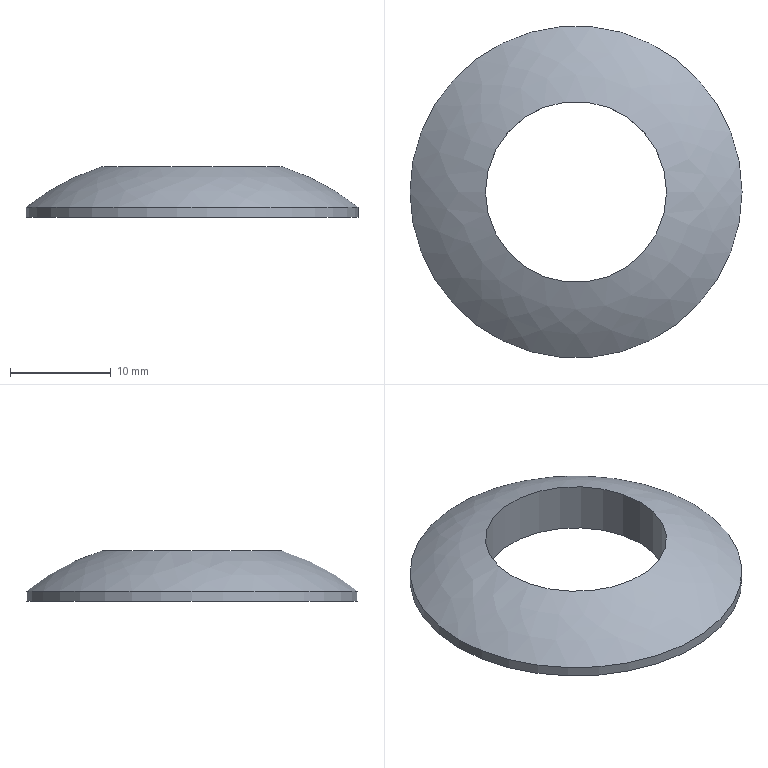Component | NX | SPHERICALWASHER2 | 1 solid | 4 faces | box 33 x 33 x 5 mm | volume 1856 mm3 | cylinder 2 | spline 1 | plane 1 | commonest cylinder face diameters 18 x1 33 x1
STEP:
#1=CARTESIAN_POINT('',(0.,0.,0.));
#2=DIRECTION('',(0.,0.,1.));
#3=DIRECTION('',(1.,0.,0.));
#4=AXIS2_PLACEMENT_3D('',#1,#2,#3);
#5=CARTESIAN_POINT('',(13.835,7.63,340.973));
#6=VERTEX_POINT('',#5);
#7=CARTESIAN_POINT('',(4.835,7.63,340.973));
#8=DIRECTION('',(0.,0.,-1.));
#9=DIRECTION('',(1.,0.,0.));
#10=AXIS2_PLACEMENT_3D('',#7,#8,#9);
#11=CIRCLE('',#10,9.);
#12=CARTESIAN_POINT('',(4.835,7.63,340.973));
#13=DIRECTION('',(0.,0.,-1.));
#14=DIRECTION('',(1.,0.,0.));
#15=AXIS2_PLACEMENT_3D('',#12,#13,#14);
#16=CYLINDRICAL_SURFACE('',#15,9.);
#17=CARTESIAN_POINT('',(0.,0.));
#18=DIRECTION('',(1.,0.));
#19=VECTOR('',#18,1.);
#20=LINE('',#17,#19);
#21=(GEOMETRIC_REPRESENTATION_CONTEXT(2)PARAMETRIC_REPRESENTATION_CONTEXT()REPRESENTATION_CONTEXT('',''));
#22=DEFINITIONAL_REPRESENTATION('',(#20),#21);
#23=PCURVE('',#16,#22);
#24=CARTESIAN_POINT('',(21.335,7.63,336.973));
#25=CARTESIAN_POINT('',(21.335,-25.37,336.973));
#26=CARTESIAN_POINT('',(-11.665,-25.37,336.973));
#27=CARTESIAN_POINT('',(-11.665,7.63,336.973));
#28=CARTESIAN_POINT('',(-11.665,40.63,336.973));
#29=CARTESIAN_POINT('',(21.335,40.63,336.973));
#30=CARTESIAN_POINT('',(21.335,7.63,336.973));
#31=CARTESIAN_POINT('',(19.087,7.63,338.746));
#32=CARTESIAN_POINT('',(19.087,-20.873,338.746));
#33=CARTESIAN_POINT('',(-9.417,-20.873,338.746));
#34=CARTESIAN_POINT('',(-9.417,7.63,338.746));
#35=CARTESIAN_POINT('',(-9.417,36.134,338.746));
#36=CARTESIAN_POINT('',(19.087,36.134,338.746));
#37=CARTESIAN_POINT('',(19.087,7.63,338.746));
#38=CARTESIAN_POINT('',(16.561,7.63,340.094));
#39=CARTESIAN_POINT('',(16.561,-15.82,340.094));
#40=CARTESIAN_POINT('',(-6.89,-15.82,340.094));
#41=CARTESIAN_POINT('',(-6.89,7.63,340.094));
#42=CARTESIAN_POINT('',(-6.89,31.081,340.094));
#43=CARTESIAN_POINT('',(16.561,31.081,340.094));
#44=CARTESIAN_POINT('',(16.561,7.63,340.094));
#45=CARTESIAN_POINT('',(13.835,7.63,340.973));
#46=CARTESIAN_POINT('',(13.835,-10.37,340.973));
#47=CARTESIAN_POINT('',(-4.165,-10.37,340.973));
#48=CARTESIAN_POINT('',(-4.165,7.63,340.973));
#49=CARTESIAN_POINT('',(-4.165,25.63,340.973));
#50=CARTESIAN_POINT('',(13.835,25.63,340.973));
#51=CARTESIAN_POINT('',(13.835,7.63,340.973));
#52=(BOUNDED_SURFACE()B_SPLINE_SURFACE(3,3,((#24,#25,#26,#27,#28,#29,#30),(#31,#32,#33,#34,#35,#36,#37),(#38,#39,#40,#41,#42,#43,#44),(#45,#46,#47,#48,#49,#50,#51)),.UNSPECIFIED.,.F.,.T.,.F.)B_SPLINE_SURFACE_WITH_KNOTS((4,4),(1,3,3,3,1),(0.,1.),(-0.5,0.,0.5,1.,1.5),.UNSPECIFIED.)GEOMETRIC_REPRESENTATION_ITEM()RATIONAL_B_SPLINE_SURFACE(((1.,0.3333,0.3333,1.,0.3333,0.3333,1.),(0.9895,0.3298,0.3298,0.9895,0.3298,0.3298,0.9895),(0.9895,0.3298,0.3298,0.9895,0.3298,0.3298,0.9895),(1.,0.3333,0.3333,1.,0.3333,0.3333,1.)))REPRESENTATION_ITEM('')SURFACE());
#53=CARTESIAN_POINT('',(1.,0.));
#54=CARTESIAN_POINT('',(1.,0.02352));
#55=CARTESIAN_POINT('',(1.,0.06491));
#56=CARTESIAN_POINT('',(1.,0.1146));
#57=CARTESIAN_POINT('',(1.,0.1575));
#58=CARTESIAN_POINT('',(1.,0.196));
#59=CARTESIAN_POINT('',(1.,0.2322));
#60=CARTESIAN_POINT('',(1.,0.2678));
#61=CARTESIAN_POINT('',(1.,0.304));
#62=CARTESIAN_POINT('',(1.,0.3425));
#63=CARTESIAN_POINT('',(1.,0.3856));
#64=CARTESIAN_POINT('',(1.,0.4343));
#65=CARTESIAN_POINT('',(1.,0.5));
#66=CARTESIAN_POINT('',(1.,0.5657));
#67=CARTESIAN_POINT('',(1.,0.6144));
#68=CARTESIAN_POINT('',(1.,0.6575));
#69=CARTESIAN_POINT('',(1.,0.696));
#70=CARTESIAN_POINT('',(1.,0.7322));
#71=CARTESIAN_POINT('',(1.,0.7678));
#72=CARTESIAN_POINT('',(1.,0.804));
#73=CARTESIAN_POINT('',(1.,0.8425));
#74=CARTESIAN_POINT('',(1.,0.8854));
#75=CARTESIAN_POINT('',(1.,0.9351));
#76=CARTESIAN_POINT('',(1.,0.9765));
#77=CARTESIAN_POINT('',(1.,1.));
#78=B_SPLINE_CURVE_WITH_KNOTS('',3,(#53,#54,#55,#56,#57,#58,#59,#60,#61,#62,#63,#64,#65,#66,#67,#68,#69,#70,#71,#72,#73,#74,#75,#76,#77),.UNSPECIFIED.,.F.,.F.,(4,1,1,1,1,1,1,1,1,1,1,1,1,1,1,1,1,1,1,1,1,1,4),(0.,0.2856,0.5712,0.8568,1.142,1.428,1.714,1.999,2.285,2.57,2.856,3.142,3.427,3.713,3.998,4.284,4.57,4.855,5.141,5.426,5.712,5.998,6.283),.QUASI_UNIFORM_KNOTS.);
#79=(GEOMETRIC_REPRESENTATION_CONTEXT(2)PARAMETRIC_REPRESENTATION_CONTEXT()REPRESENTATION_CONTEXT('',''));
#80=DEFINITIONAL_REPRESENTATION('',(#78),#79);
#81=PCURVE('',#52,#80);
#82=SURFACE_CURVE('',#11,(#23,#81),.PCURVE_S1.);
#83=EDGE_CURVE('',#6,#6,#82,.T.);
#84=ORIENTED_EDGE('',*,*,#83,.T.);
#85=CARTESIAN_POINT('',(13.835,7.63,335.973));
#86=VERTEX_POINT('',#85);
#87=CARTESIAN_POINT('',(13.835,7.63,340.973));
#88=CARTESIAN_POINT('',(13.835,7.63,335.973));
#89=B_SPLINE_CURVE_WITH_KNOTS('',1,(#87,#88),.UNSPECIFIED.,.F.,.F.,(2,2),(0.,5.),.PIECEWISE_BEZIER_KNOTS.);
#90=CARTESIAN_POINT('',(6.283,0.));
#91=DIRECTION('',(0.,1.));
#92=VECTOR('',#91,1.);
#93=LINE('',#90,#92);
#94=(GEOMETRIC_REPRESENTATION_CONTEXT(2)PARAMETRIC_REPRESENTATION_CONTEXT()REPRESENTATION_CONTEXT('',''));
#95=DEFINITIONAL_REPRESENTATION('',(#93),#94);
#96=PCURVE('',#16,#95);
#97=CARTESIAN_POINT('',(0.,0.));
#98=DIRECTION('',(0.,1.));
#99=VECTOR('',#98,1.);
#100=LINE('',#97,#99);
#101=(GEOMETRIC_REPRESENTATION_CONTEXT(2)PARAMETRIC_REPRESENTATION_CONTEXT()REPRESENTATION_CONTEXT('',''));
#102=DEFINITIONAL_REPRESENTATION('',(#100),#101);
#103=PCURVE('',#16,#102);
#104=SEAM_CURVE('',#89,(#96,#103),.PCURVE_S1.);
#105=EDGE_CURVE('',#6,#86,#104,.T.);
#106=ORIENTED_EDGE('',*,*,#105,.T.);
#107=CARTESIAN_POINT('',(4.835,7.63,335.973));
#108=DIRECTION('',(0.,0.,-1.));
#109=DIRECTION('',(1.,0.,0.));
#110=AXIS2_PLACEMENT_3D('',#107,#108,#109);
#111=CIRCLE('',#110,9.);
#112=CARTESIAN_POINT('',(0.,5.));
#113=DIRECTION('',(1.,0.));
#114=VECTOR('',#113,1.);
#115=LINE('',#112,#114);
#116=(GEOMETRIC_REPRESENTATION_CONTEXT(2)PARAMETRIC_REPRESENTATION_CONTEXT()REPRESENTATION_CONTEXT('',''));
#117=DEFINITIONAL_REPRESENTATION('',(#115),#116);
#118=PCURVE('',#16,#117);
#119=CARTESIAN_POINT('',(-11.665,7.63,335.973));
#120=DIRECTION('',(0.,0.,1.));
#121=DIRECTION('',(-1.,0.,0.));
#122=AXIS2_PLACEMENT_3D('',#119,#120,#121);
#123=PLANE('',#122);
#124=CARTESIAN_POINT('',(-25.5,0.));
#125=CARTESIAN_POINT('',(-25.5,15.588));
#126=CARTESIAN_POINT('',(-12.,7.794));
#127=CARTESIAN_POINT('',(1.5,0.));
#128=CARTESIAN_POINT('',(-12.,-7.794));
#129=CARTESIAN_POINT('',(-25.5,-15.588));
#130=CARTESIAN_POINT('',(-25.5,0.));
#131=(BOUNDED_CURVE()B_SPLINE_CURVE(2,(#124,#125,#126,#127,#128,#129,#130),.UNSPECIFIED.,.T.,.F.)B_SPLINE_CURVE_WITH_KNOTS((1,2,2,2,2,1),(-2.094,0.,2.094,4.189,6.283,8.378),.UNSPECIFIED.)CURVE()GEOMETRIC_REPRESENTATION_ITEM()RATIONAL_B_SPLINE_CURVE((1.,0.5,1.,0.5,1.,0.5,1.))REPRESENTATION_ITEM(''));
#132=(GEOMETRIC_REPRESENTATION_CONTEXT(2)PARAMETRIC_REPRESENTATION_CONTEXT()REPRESENTATION_CONTEXT('',''));
#133=DEFINITIONAL_REPRESENTATION('',(#131),#132);
#134=PCURVE('',#123,#133);
#135=SURFACE_CURVE('',#111,(#118,#134),.PCURVE_S1.);
#136=EDGE_CURVE('',#86,#86,#135,.T.);
#137=ORIENTED_EDGE('',*,*,#136,.F.);
#138=ORIENTED_EDGE('',*,*,#105,.F.);
#139=EDGE_LOOP('',(#84,#106,#137,#138));
#140=FACE_BOUND('',#139,.F.);
#141=ADVANCED_FACE('',(#140),#16,.F.);
#142=CARTESIAN_POINT('',(21.335,7.63,336.973));
#143=VERTEX_POINT('',#142);
#144=CARTESIAN_POINT('',(4.835,7.63,336.973));
#145=DIRECTION('',(0.,0.,-1.));
#146=DIRECTION('',(1.,0.,0.));
#147=AXIS2_PLACEMENT_3D('',#144,#145,#146);
#148=CIRCLE('',#147,16.5);
#149=CARTESIAN_POINT('',(0.,0.));
#150=CARTESIAN_POINT('',(0.,0.02352));
#151=CARTESIAN_POINT('',(0.,0.06491));
#152=CARTESIAN_POINT('',(0.,0.1146));
#153=CARTESIAN_POINT('',(0.,0.1575));
#154=CARTESIAN_POINT('',(0.,0.196));
#155=CARTESIAN_POINT('',(0.,0.2322));
#156=CARTESIAN_POINT('',(0.,0.2678));
#157=CARTESIAN_POINT('',(0.,0.304));
#158=CARTESIAN_POINT('',(0.,0.3425));
#159=CARTESIAN_POINT('',(0.,0.3856));
#160=CARTESIAN_POINT('',(0.,0.4343));
#161=CARTESIAN_POINT('',(0.,0.5));
#162=CARTESIAN_POINT('',(0.,0.5657));
#163=CARTESIAN_POINT('',(0.,0.6144));
#164=CARTESIAN_POINT('',(0.,0.6575));
#165=CARTESIAN_POINT('',(0.,0.696));
#166=CARTESIAN_POINT('',(0.,0.7322));
#167=CARTESIAN_POINT('',(0.,0.7678));
#168=CARTESIAN_POINT('',(0.,0.804));
#169=CARTESIAN_POINT('',(0.,0.8425));
#170=CARTESIAN_POINT('',(0.,0.8854));
#171=CARTESIAN_POINT('',(0.,0.9351));
#172=CARTESIAN_POINT('',(0.,0.9765));
#173=CARTESIAN_POINT('',(0.,1.));
#174=B_SPLINE_CURVE_WITH_KNOTS('',3,(#149,#150,#151,#152,#153,#154,#155,#156,#157,#158,#159,#160,#161,#162,#163,#164,#165,#166,#167,#168,#169,#170,#171,#172,#173),.UNSPECIFIED.,.F.,.F.,(4,1,1,1,1,1,1,1,1,1,1,1,1,1,1,1,1,1,1,1,1,1,4),(0.,0.2856,0.5712,0.8568,1.142,1.428,1.714,1.999,2.285,2.57,2.856,3.142,3.427,3.713,3.998,4.284,4.57,4.855,5.141,5.426,5.712,5.998,6.283),.QUASI_UNIFORM_KNOTS.);
#175=(GEOMETRIC_REPRESENTATION_CONTEXT(2)PARAMETRIC_REPRESENTATION_CONTEXT()REPRESENTATION_CONTEXT('',''));
#176=DEFINITIONAL_REPRESENTATION('',(#174),#175);
#177=PCURVE('',#52,#176);
#178=CARTESIAN_POINT('',(4.835,7.63,340.973));
#179=DIRECTION('',(0.,0.,-1.));
#180=DIRECTION('',(1.,0.,0.));
#181=AXIS2_PLACEMENT_3D('',#178,#179,#180);
#182=CYLINDRICAL_SURFACE('',#181,16.5);
#183=CARTESIAN_POINT('',(0.,4.));
#184=DIRECTION('',(1.,0.));
#185=VECTOR('',#184,1.);
#186=LINE('',#183,#185);
#187=(GEOMETRIC_REPRESENTATION_CONTEXT(2)PARAMETRIC_REPRESENTATION_CONTEXT()REPRESENTATION_CONTEXT('',''));
#188=DEFINITIONAL_REPRESENTATION('',(#186),#187);
#189=PCURVE('',#182,#188);
#190=SURFACE_CURVE('',#148,(#177,#189),.PCURVE_S1.);
#191=EDGE_CURVE('',#143,#143,#190,.T.);
#192=ORIENTED_EDGE('',*,*,#191,.F.);
#193=CARTESIAN_POINT('',(21.335,7.63,336.973));
#194=CARTESIAN_POINT('',(19.087,7.63,338.746));
#195=CARTESIAN_POINT('',(16.561,7.63,340.094));
#196=CARTESIAN_POINT('',(13.835,7.63,340.973));
#197=(BOUNDED_CURVE()B_SPLINE_CURVE(3,(#193,#194,#195,#196),.UNSPECIFIED.,.F.,.F.)B_SPLINE_CURVE_WITH_KNOTS((4,4),(0.,1.),.PIECEWISE_BEZIER_KNOTS.)CURVE()GEOMETRIC_REPRESENTATION_ITEM()RATIONAL_B_SPLINE_CURVE((1.,0.9895,0.9895,1.))REPRESENTATION_ITEM(''));
#198=CARTESIAN_POINT('',(0.,0.));
#199=DIRECTION('',(1.,0.));
#200=VECTOR('',#199,1.);
#201=LINE('',#198,#200);
#202=(GEOMETRIC_REPRESENTATION_CONTEXT(2)PARAMETRIC_REPRESENTATION_CONTEXT()REPRESENTATION_CONTEXT('',''));
#203=DEFINITIONAL_REPRESENTATION('',(#201),#202);
#204=PCURVE('',#52,#203);
#205=CARTESIAN_POINT('',(0.,1.));
#206=DIRECTION('',(1.,0.));
#207=VECTOR('',#206,1.);
#208=LINE('',#205,#207);
#209=(GEOMETRIC_REPRESENTATION_CONTEXT(2)PARAMETRIC_REPRESENTATION_CONTEXT()REPRESENTATION_CONTEXT('',''));
#210=DEFINITIONAL_REPRESENTATION('',(#208),#209);
#211=PCURVE('',#52,#210);
#212=SEAM_CURVE('',#197,(#204,#211),.PCURVE_S1.);
#213=EDGE_CURVE('',#143,#6,#212,.T.);
#214=ORIENTED_EDGE('',*,*,#213,.T.);
#215=ORIENTED_EDGE('',*,*,#83,.T.);
#216=ORIENTED_EDGE('',*,*,#213,.F.);
#217=EDGE_LOOP('',(#192,#214,#215,#216));
#218=FACE_BOUND('',#217,.T.);
#219=ADVANCED_FACE('',(#218),#52,.T.);
#220=CARTESIAN_POINT('',(21.335,7.63,335.973));
#221=VERTEX_POINT('',#220);
#222=CARTESIAN_POINT('',(4.835,7.63,335.973));
#223=DIRECTION('',(0.,0.,-1.));
#224=DIRECTION('',(1.,0.,0.));
#225=AXIS2_PLACEMENT_3D('',#222,#223,#224);
#226=CIRCLE('',#225,16.5);
#227=CARTESIAN_POINT('',(0.,5.));
#228=DIRECTION('',(1.,0.));
#229=VECTOR('',#228,1.);
#230=LINE('',#227,#229);
#231=(GEOMETRIC_REPRESENTATION_CONTEXT(2)PARAMETRIC_REPRESENTATION_CONTEXT()REPRESENTATION_CONTEXT('',''));
#232=DEFINITIONAL_REPRESENTATION('',(#230),#231);
#233=PCURVE('',#182,#232);
#234=CARTESIAN_POINT('',(-33.,0.));
#235=CARTESIAN_POINT('',(-33.,28.579));
#236=CARTESIAN_POINT('',(-8.25,14.289));
#237=CARTESIAN_POINT('',(16.5,0.));
#238=CARTESIAN_POINT('',(-8.25,-14.289));
#239=CARTESIAN_POINT('',(-33.,-28.579));
#240=CARTESIAN_POINT('',(-33.,0.));
#241=(BOUNDED_CURVE()B_SPLINE_CURVE(2,(#234,#235,#236,#237,#238,#239,#240),.UNSPECIFIED.,.T.,.F.)B_SPLINE_CURVE_WITH_KNOTS((1,2,2,2,2,1),(-2.094,0.,2.094,4.189,6.283,8.378),.UNSPECIFIED.)CURVE()GEOMETRIC_REPRESENTATION_ITEM()RATIONAL_B_SPLINE_CURVE((1.,0.5,1.,0.5,1.,0.5,1.))REPRESENTATION_ITEM(''));
#242=(GEOMETRIC_REPRESENTATION_CONTEXT(2)PARAMETRIC_REPRESENTATION_CONTEXT()REPRESENTATION_CONTEXT('',''));
#243=DEFINITIONAL_REPRESENTATION('',(#241),#242);
#244=PCURVE('',#123,#243);
#245=SURFACE_CURVE('',#226,(#233,#244),.PCURVE_S1.);
#246=EDGE_CURVE('',#221,#221,#245,.T.);
#247=ORIENTED_EDGE('',*,*,#246,.F.);
#248=CARTESIAN_POINT('',(21.335,7.63,336.973));
#249=CARTESIAN_POINT('',(21.335,7.63,335.973));
#250=B_SPLINE_CURVE_WITH_KNOTS('',1,(#248,#249),.UNSPECIFIED.,.F.,.F.,(2,2),(4.,5.),.PIECEWISE_BEZIER_KNOTS.);
#251=CARTESIAN_POINT('',(0.,0.));
#252=DIRECTION('',(0.,1.));
#253=VECTOR('',#252,1.);
#254=LINE('',#251,#253);
#255=(GEOMETRIC_REPRESENTATION_CONTEXT(2)PARAMETRIC_REPRESENTATION_CONTEXT()REPRESENTATION_CONTEXT('',''));
#256=DEFINITIONAL_REPRESENTATION('',(#254),#255);
#257=PCURVE('',#182,#256);
#258=CARTESIAN_POINT('',(6.283,0.));
#259=DIRECTION('',(0.,1.));
#260=VECTOR('',#259,1.);
#261=LINE('',#258,#260);
#262=(GEOMETRIC_REPRESENTATION_CONTEXT(2)PARAMETRIC_REPRESENTATION_CONTEXT()REPRESENTATION_CONTEXT('',''));
#263=DEFINITIONAL_REPRESENTATION('',(#261),#262);
#264=PCURVE('',#182,#263);
#265=SEAM_CURVE('',#250,(#257,#264),.PCURVE_S1.);
#266=EDGE_CURVE('',#143,#221,#265,.T.);
#267=ORIENTED_EDGE('',*,*,#266,.F.);
#268=ORIENTED_EDGE('',*,*,#191,.T.);
#269=ORIENTED_EDGE('',*,*,#266,.T.);
#270=EDGE_LOOP('',(#247,#267,#268,#269));
#271=FACE_BOUND('',#270,.T.);
#272=ADVANCED_FACE('',(#271),#182,.T.);
#273=ORIENTED_EDGE('',*,*,#136,.F.);
#274=EDGE_LOOP('',(#273));
#275=FACE_BOUND('',#274,.T.);
#276=ORIENTED_EDGE('',*,*,#246,.T.);
#277=EDGE_LOOP('',(#276));
#278=FACE_BOUND('',#277,.T.);
#279=ADVANCED_FACE('',(#275,#278),#123,.F.);
#280=CLOSED_SHELL('',(#141,#219,#272,#279));
#281=MANIFOLD_SOLID_BREP('',#280);
#282=(LENGTH_UNIT()NAMED_UNIT(*)SI_UNIT(.MILLI.,.METRE.));
#283=UNCERTAINTY_MEASURE_WITH_UNIT(LENGTH_MEASURE(0.00001),#282,'','');
#284=(NAMED_UNIT(*)PLANE_ANGLE_UNIT()SI_UNIT($,.RADIAN.));
#285=(NAMED_UNIT(*)SI_UNIT($,.STERADIAN.)SOLID_ANGLE_UNIT());
#286=(GEOMETRIC_REPRESENTATION_CONTEXT(3)GLOBAL_UNCERTAINTY_ASSIGNED_CONTEXT((#283))GLOBAL_UNIT_ASSIGNED_CONTEXT((#282,#284,#285))REPRESENTATION_CONTEXT('',''));
#287=ADVANCED_BREP_SHAPE_REPRESENTATION('',(#4,#281),#286);